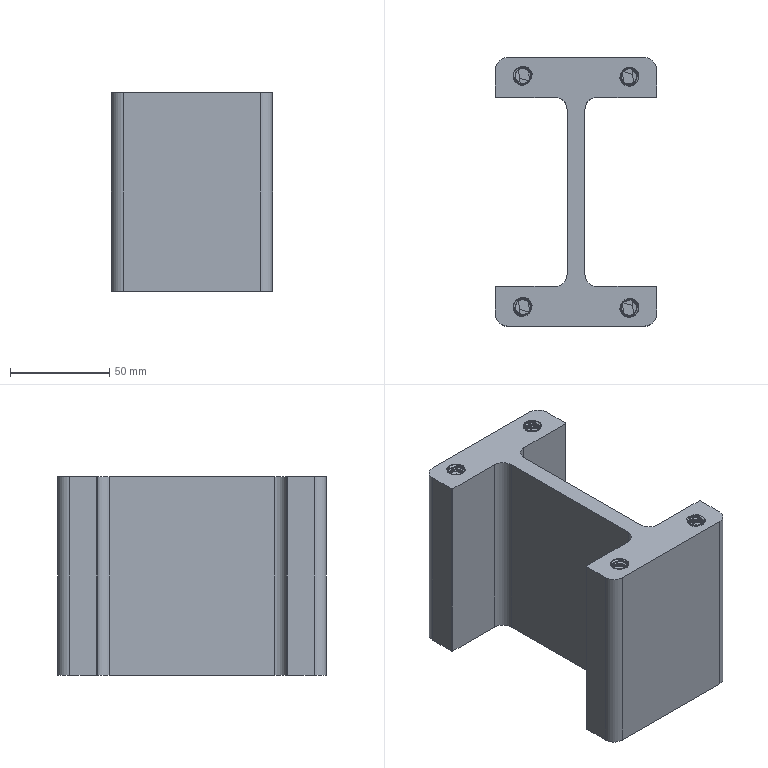Component | NX | PUNCH | 1 solid | 54 faces | volume 401036 mm3 | plane 22 | cylinder 20 | spline 12 | commonest cylinder face diameters 8 x4 12 x4 1 x4 11.8 x4 10 x4